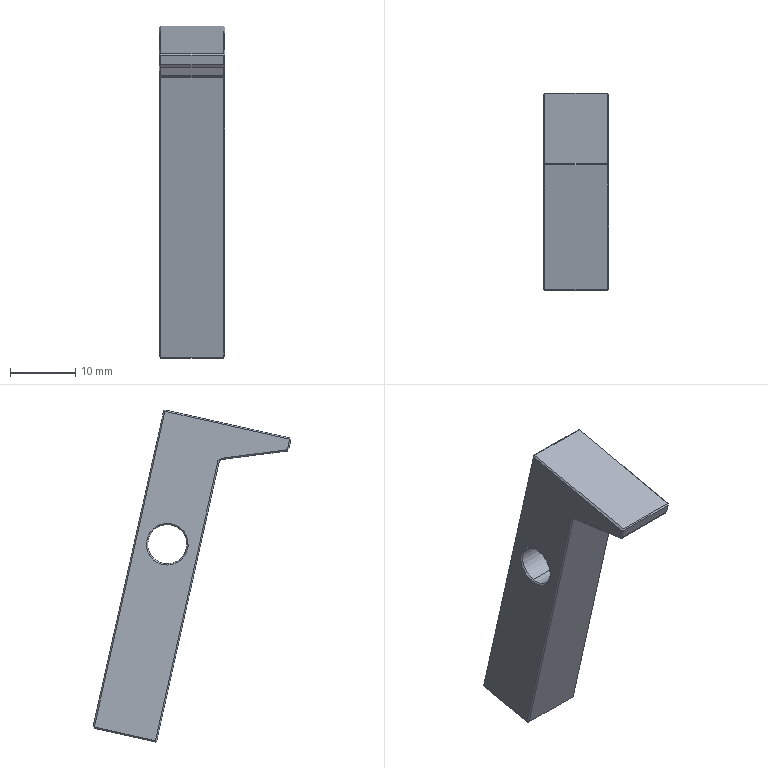Component | SolidWorks | PressJaw-1 | 1 solid | 44 faces | box 10 x 30.33 x 50.89 mm | volume 5092 mm3 | plane 36 | cone 4 | cylinder 2 | spline 2 | commonest cylinder face diameters 6 x2 | material 45
STEP:
#1=COLOUR_RGB('',0.7922,0.8196,0.9333);
#2=FILL_AREA_STYLE_COLOUR('',#1);
#3=FILL_AREA_STYLE('',(#2));
#4=SURFACE_STYLE_FILL_AREA(#3);
#5=SURFACE_SIDE_STYLE('',(#4));
#6=SURFACE_STYLE_USAGE(.BOTH.,#5);
#7=PRESENTATION_STYLE_ASSIGNMENT((#6));
#8=CARTESIAN_POINT('',(-14.809,1.597,40.726));
#9=VERTEX_POINT('',#8);
#10=CARTESIAN_POINT('',(-14.809,1.546,40.957));
#11=VERTEX_POINT('',#10);
#12=CARTESIAN_POINT('',(-14.809,1.571,40.842));
#13=DIRECTION('',(-1.,0.,0.));
#14=DIRECTION('',(0.,0.218,-0.9759));
#15=AXIS2_PLACEMENT_3D('',#12,#13,#14);
#16=CIRCLE('',#15,0.1181);
#17=EDGE_CURVE('',#9,#11,#16,.T.);
#18=ORIENTED_EDGE('',*,*,#17,.F.);
#19=CARTESIAN_POINT('',(-14.817,1.599,40.719));
#20=VERTEX_POINT('',#19);
#21=CARTESIAN_POINT('',(-14.809,1.597,40.726));
#22=DIRECTION('',(-0.7071,0.1542,-0.6901));
#23=VECTOR('',#22,39.37);
#24=LINE('',#21,#23);
#25=EDGE_CURVE('',#9,#20,#24,.T.);
#26=ORIENTED_EDGE('',*,*,#25,.T.);
#27=CARTESIAN_POINT('',(-14.817,1.544,40.965));
#28=VERTEX_POINT('',#27);
#29=CARTESIAN_POINT('',(-14.817,1.571,40.842));
#30=DIRECTION('',(1.,-0.,-0.));
#31=DIRECTION('',(0.,0.218,-0.9759));
#32=AXIS2_PLACEMENT_3D('',#29,#30,#31);
#33=CIRCLE('',#32,0.126);
#34=EDGE_CURVE('',#28,#20,#33,.T.);
#35=ORIENTED_EDGE('',*,*,#34,.F.);
#36=CARTESIAN_POINT('',(-14.809,1.546,40.957));
#37=DIRECTION('',(-0.7071,-0.1542,0.6901));
#38=VECTOR('',#37,39.37);
#39=LINE('',#36,#38);
#40=EDGE_CURVE('',#11,#28,#39,.T.);
#41=ORIENTED_EDGE('',*,*,#40,.F.);
#42=EDGE_LOOP('',(#18,#26,#35,#41));
#43=FACE_OUTER_BOUND('',#42,.T.);
#44=CARTESIAN_POINT('',(-14.809,1.571,40.842));
#45=DIRECTION('',(-1.,0.,0.));
#46=DIRECTION('',(0.,-0.218,0.9759));
#47=AXIS2_PLACEMENT_3D('',#44,#45,#46);
#48=CONICAL_SURFACE('',#47,0.1181,0.7854);
#49=ADVANCED_FACE('',(#43),#48,.F.);
#50=CARTESIAN_POINT('',(-14.431,1.546,40.957));
#51=VERTEX_POINT('',#50);
#52=CARTESIAN_POINT('',(-14.431,1.597,40.726));
#53=VERTEX_POINT('',#52);
#54=CARTESIAN_POINT('',(-14.431,1.571,40.842));
#55=DIRECTION('',(1.,-0.,-0.));
#56=DIRECTION('',(0.,0.218,-0.9759));
#57=AXIS2_PLACEMENT_3D('',#54,#55,#56);
#58=CIRCLE('',#57,0.1181);
#59=EDGE_CURVE('',#51,#53,#58,.T.);
#60=ORIENTED_EDGE('',*,*,#59,.F.);
#61=CARTESIAN_POINT('',(-14.424,1.544,40.965));
#62=VERTEX_POINT('',#61);
#63=CARTESIAN_POINT('',(-14.424,1.544,40.965));
#64=DIRECTION('',(0.7071,-0.1542,0.6901));
#65=VECTOR('',#64,39.37);
#66=LINE('',#63,#65);
#67=EDGE_CURVE('',#51,#62,#66,.T.);
#68=ORIENTED_EDGE('',*,*,#67,.T.);
#69=CARTESIAN_POINT('',(-14.424,1.599,40.719));
#70=VERTEX_POINT('',#69);
#71=CARTESIAN_POINT('',(-14.424,1.571,40.842));
#72=DIRECTION('',(-1.,0.,0.));
#73=DIRECTION('',(0.,0.218,-0.9759));
#74=AXIS2_PLACEMENT_3D('',#71,#72,#73);
#75=CIRCLE('',#74,0.126);
#76=EDGE_CURVE('',#70,#62,#75,.T.);
#77=ORIENTED_EDGE('',*,*,#76,.F.);
#78=CARTESIAN_POINT('',(-14.424,1.599,40.719));
#79=DIRECTION('',(0.7071,0.1542,-0.6901));
#80=VECTOR('',#79,39.37);
#81=LINE('',#78,#80);
#82=EDGE_CURVE('',#53,#70,#81,.T.);
#83=ORIENTED_EDGE('',*,*,#82,.F.);
#84=EDGE_LOOP('',(#60,#68,#77,#83));
#85=FACE_OUTER_BOUND('',#84,.T.);
#86=CARTESIAN_POINT('',(-14.424,1.571,40.842));
#87=DIRECTION('',(1.,-0.,-0.));
#88=DIRECTION('',(0.,0.218,-0.9759));
#89=AXIS2_PLACEMENT_3D('',#86,#87,#88);
#90=CONICAL_SURFACE('',#89,0.126,0.7854);
#91=ADVANCED_FACE('',(#85),#90,.F.);
#92=ORIENTED_EDGE('',*,*,#17,.T.);
#93=CARTESIAN_POINT('',(-14.817,1.546,40.957));
#94=DIRECTION('',(1.,-0.,-0.));
#95=VECTOR('',#94,39.37);
#96=LINE('',#93,#95);
#97=EDGE_CURVE('',#11,#51,#96,.T.);
#98=ORIENTED_EDGE('',*,*,#97,.T.);
#99=ORIENTED_EDGE('',*,*,#59,.T.);
#100=CARTESIAN_POINT('',(-14.817,1.597,40.726));
#101=DIRECTION('',(1.,-0.,-0.));
#102=VECTOR('',#101,39.37);
#103=LINE('',#100,#102);
#104=EDGE_CURVE('',#9,#53,#103,.T.);
#105=ORIENTED_EDGE('',*,*,#104,.F.);
#106=EDGE_LOOP('',(#92,#98,#99,#105));
#107=FACE_OUTER_BOUND('',#106,.T.);
#108=CARTESIAN_POINT('',(-14.817,1.571,40.842));
#109=DIRECTION('',(1.,-0.,-0.));
#110=DIRECTION('',(0.,0.218,-0.9759));
#111=AXIS2_PLACEMENT_3D('',#108,#109,#110);
#112=CYLINDRICAL_SURFACE('',#111,0.1181);
#113=ADVANCED_FACE('',(#107),#112,.F.);
#114=CARTESIAN_POINT('',(-14.817,1.244,41.36));
#115=VERTEX_POINT('',#114);
#116=CARTESIAN_POINT('',(-14.817,0.8471,41.412));
#117=VERTEX_POINT('',#116);
#118=CARTESIAN_POINT('',(-14.817,2.216,41.234));
#119=DIRECTION('',(-0.,-0.9917,0.1289));
#120=VECTOR('',#119,39.37);
#121=LINE('',#118,#120);
#122=EDGE_CURVE('',#115,#117,#121,.T.);
#123=ORIENTED_EDGE('',*,*,#122,.T.);
#124=CARTESIAN_POINT('',(-14.817,0.8328,41.475));
#125=VERTEX_POINT('',#124);
#126=CARTESIAN_POINT('',(-14.817,1.26,39.562));
#127=DIRECTION('',(0.,-0.218,0.9759));
#128=VECTOR('',#127,39.37);
#129=LINE('',#126,#128);
#130=EDGE_CURVE('',#117,#125,#129,.T.);
#131=ORIENTED_EDGE('',*,*,#130,.T.);
#132=CARTESIAN_POINT('',(-14.817,1.586,41.644));
#133=VERTEX_POINT('',#132);
#134=CARTESIAN_POINT('',(-14.817,1.594,41.645));
#135=DIRECTION('',(0.,0.9759,0.218));
#136=VECTOR('',#135,39.37);
#137=LINE('',#134,#136);
#138=EDGE_CURVE('',#125,#133,#137,.T.);
#139=ORIENTED_EDGE('',*,*,#138,.T.);
#140=CARTESIAN_POINT('',(-14.817,2.012,39.738));
#141=VERTEX_POINT('',#140);
#142=CARTESIAN_POINT('',(-14.817,2.013,39.73));
#143=DIRECTION('',(-0.,0.218,-0.9759));
#144=VECTOR('',#143,39.37);
#145=LINE('',#142,#144);
#146=EDGE_CURVE('',#133,#141,#145,.T.);
#147=ORIENTED_EDGE('',*,*,#146,.T.);
#148=CARTESIAN_POINT('',(-14.817,1.643,39.655));
#149=VERTEX_POINT('',#148);
#150=CARTESIAN_POINT('',(-14.817,2.019,39.74));
#151=DIRECTION('',(-0.,-0.9759,-0.218));
#152=VECTOR('',#151,39.37);
#153=LINE('',#150,#152);
#154=EDGE_CURVE('',#141,#149,#153,.T.);
#155=ORIENTED_EDGE('',*,*,#154,.T.);
#156=CARTESIAN_POINT('',(-14.817,1.265,41.344));
#157=VERTEX_POINT('',#156);
#158=CARTESIAN_POINT('',(-14.817,1.645,39.648));
#159=DIRECTION('',(0.,-0.218,0.9759));
#160=VECTOR('',#159,39.37);
#161=LINE('',#158,#160);
#162=EDGE_CURVE('',#149,#157,#161,.T.);
#163=ORIENTED_EDGE('',*,*,#162,.T.);
#164=CARTESIAN_POINT('',(-14.817,1.244,41.36));
#165=CARTESIAN_POINT('',(-14.817,1.265,41.344));
#166=B_SPLINE_CURVE_WITH_KNOTS('',1,(#164,#165),.UNSPECIFIED.,.F.,.F.,(2,2),(0.,0.0006718),.UNSPECIFIED.);
#167=EDGE_CURVE('',#115,#157,#166,.T.);
#168=ORIENTED_EDGE('',*,*,#167,.F.);
#169=EDGE_LOOP('',(#123,#131,#139,#147,#155,#163,#168));
#170=FACE_OUTER_BOUND('',#169,.T.);
#171=ORIENTED_EDGE('',*,*,#34,.T.);
#172=CARTESIAN_POINT('',(-14.817,1.571,40.842));
#173=DIRECTION('',(1.,-0.,-0.));
#174=DIRECTION('',(0.,0.218,-0.9759));
#175=AXIS2_PLACEMENT_3D('',#172,#173,#174);
#176=CIRCLE('',#175,0.126);
#177=EDGE_CURVE('',#20,#28,#176,.T.);
#178=ORIENTED_EDGE('',*,*,#177,.T.);
#179=EDGE_LOOP('',(#171,#178));
#180=FACE_BOUND('',#179,.T.);
#181=CARTESIAN_POINT('',(-14.817,2.021,39.732));
#182=DIRECTION('',(1.,-0.,-0.));
#183=DIRECTION('',(-0.,0.218,-0.9759));
#184=AXIS2_PLACEMENT_3D('',#181,#182,#183);
#185=PLANE('',#184);
#186=ADVANCED_FACE('',(#170,#180),#185,.F.);
#187=CARTESIAN_POINT('',(-14.424,2.012,39.738));
#188=VERTEX_POINT('',#187);
#189=CARTESIAN_POINT('',(-14.424,1.586,41.644));
#190=VERTEX_POINT('',#189);
#191=CARTESIAN_POINT('',(-14.424,1.584,41.651));
#192=DIRECTION('',(0.,-0.218,0.9759));
#193=VECTOR('',#192,39.37);
#194=LINE('',#191,#193);
#195=EDGE_CURVE('',#188,#190,#194,.T.);
#196=ORIENTED_EDGE('',*,*,#195,.T.);
#197=CARTESIAN_POINT('',(-14.424,0.8328,41.475));
#198=VERTEX_POINT('',#197);
#199=CARTESIAN_POINT('',(-14.424,0.8251,41.474));
#200=DIRECTION('',(-0.,-0.9759,-0.218));
#201=VECTOR('',#200,39.37);
#202=LINE('',#199,#201);
#203=EDGE_CURVE('',#190,#198,#202,.T.);
#204=ORIENTED_EDGE('',*,*,#203,.T.);
#205=CARTESIAN_POINT('',(-14.424,0.8471,41.412));
#206=VERTEX_POINT('',#205);
#207=CARTESIAN_POINT('',(-14.424,0.8483,41.406));
#208=DIRECTION('',(-0.,0.218,-0.9759));
#209=VECTOR('',#208,39.37);
#210=LINE('',#207,#209);
#211=EDGE_CURVE('',#198,#206,#210,.T.);
#212=ORIENTED_EDGE('',*,*,#211,.T.);
#213=CARTESIAN_POINT('',(-14.424,1.244,41.36));
#214=VERTEX_POINT('',#213);
#215=CARTESIAN_POINT('',(-14.424,1.257,41.358));
#216=DIRECTION('',(0.,0.9917,-0.1289));
#217=VECTOR('',#216,39.37);
#218=LINE('',#215,#217);
#219=EDGE_CURVE('',#206,#214,#218,.T.);
#220=ORIENTED_EDGE('',*,*,#219,.T.);
#221=CARTESIAN_POINT('',(-14.424,1.265,41.344));
#222=VERTEX_POINT('',#221);
#223=CARTESIAN_POINT('',(-14.424,1.265,41.344));
#224=CARTESIAN_POINT('',(-14.424,1.244,41.36));
#225=B_SPLINE_CURVE_WITH_KNOTS('',1,(#223,#224),.UNSPECIFIED.,.F.,.F.,(2,2),(0.,0.0006718),.UNSPECIFIED.);
#226=EDGE_CURVE('',#222,#214,#225,.T.);
#227=ORIENTED_EDGE('',*,*,#226,.F.);
#228=CARTESIAN_POINT('',(-14.424,1.643,39.655));
#229=VERTEX_POINT('',#228);
#230=CARTESIAN_POINT('',(-14.424,1.645,39.648));
#231=DIRECTION('',(-0.,0.218,-0.9759));
#232=VECTOR('',#231,39.37);
#233=LINE('',#230,#232);
#234=EDGE_CURVE('',#222,#229,#233,.T.);
#235=ORIENTED_EDGE('',*,*,#234,.T.);
#236=CARTESIAN_POINT('',(-14.424,2.019,39.74));
#237=DIRECTION('',(0.,0.9759,0.218));
#238=VECTOR('',#237,39.37);
#239=LINE('',#236,#238);
#240=EDGE_CURVE('',#229,#188,#239,.T.);
#241=ORIENTED_EDGE('',*,*,#240,.T.);
#242=EDGE_LOOP('',(#196,#204,#212,#220,#227,#235,#241));
#243=FACE_OUTER_BOUND('',#242,.T.);
#244=ORIENTED_EDGE('',*,*,#76,.T.);
#245=CARTESIAN_POINT('',(-14.424,1.571,40.842));
#246=DIRECTION('',(-1.,0.,0.));
#247=DIRECTION('',(0.,0.218,-0.9759));
#248=AXIS2_PLACEMENT_3D('',#245,#246,#247);
#249=CIRCLE('',#248,0.126);
#250=EDGE_CURVE('',#62,#70,#249,.T.);
#251=ORIENTED_EDGE('',*,*,#250,.T.);
#252=EDGE_LOOP('',(#244,#251));
#253=FACE_BOUND('',#252,.T.);
#254=CARTESIAN_POINT('',(-14.424,2.021,39.732));
#255=DIRECTION('',(1.,-0.,-0.));
#256=DIRECTION('',(-0.,0.218,-0.9759));
#257=AXIS2_PLACEMENT_3D('',#254,#255,#256);
#258=PLANE('',#257);
#259=ADVANCED_FACE('',(#243,#253),#258,.T.);
#260=CARTESIAN_POINT('',(-14.809,1.645,39.648));
#261=VERTEX_POINT('',#260);
#262=CARTESIAN_POINT('',(-14.809,2.013,39.73));
#263=VERTEX_POINT('',#262);
#264=CARTESIAN_POINT('',(-14.809,1.637,39.646));
#265=DIRECTION('',(0.,0.9759,0.218));
#266=VECTOR('',#265,39.37);
#267=LINE('',#264,#266);
#268=EDGE_CURVE('',#261,#263,#267,.T.);
#269=ORIENTED_EDGE('',*,*,#268,.T.);
#270=CARTESIAN_POINT('',(-14.431,2.013,39.73));
#271=VERTEX_POINT('',#270);
#272=CARTESIAN_POINT('',(-14.817,2.013,39.73));
#273=DIRECTION('',(1.,-0.,-0.));
#274=VECTOR('',#273,39.37);
#275=LINE('',#272,#274);
#276=EDGE_CURVE('',#263,#271,#275,.T.);
#277=ORIENTED_EDGE('',*,*,#276,.T.);
#278=CARTESIAN_POINT('',(-14.431,1.645,39.648));
#279=VERTEX_POINT('',#278);
#280=CARTESIAN_POINT('',(-14.431,1.637,39.646));
#281=DIRECTION('',(-0.,-0.9759,-0.218));
#282=VECTOR('',#281,39.37);
#283=LINE('',#280,#282);
#284=EDGE_CURVE('',#271,#279,#283,.T.);
#285=ORIENTED_EDGE('',*,*,#284,.T.);
#286=CARTESIAN_POINT('',(-14.817,1.645,39.648));
#287=DIRECTION('',(-1.,0.,0.));
#288=VECTOR('',#287,39.37);
#289=LINE('',#286,#288);
#290=EDGE_CURVE('',#279,#261,#289,.T.);
#291=ORIENTED_EDGE('',*,*,#290,.T.);
#292=EDGE_LOOP('',(#269,#277,#285,#291));
#293=FACE_OUTER_BOUND('',#292,.T.);
#294=CARTESIAN_POINT('',(-14.817,1.637,39.646));
#295=DIRECTION('',(0.,-0.218,0.9759));
#296=DIRECTION('',(1.,-0.,-0.));
#297=AXIS2_PLACEMENT_3D('',#294,#295,#296);
#298=PLANE('',#297);
#299=ADVANCED_FACE('',(#293),#298,.F.);
#300=CARTESIAN_POINT('',(-14.431,1.635,39.654));
#301=VERTEX_POINT('',#300);
#302=CARTESIAN_POINT('',(-14.431,1.258,41.343));
#303=VERTEX_POINT('',#302);
#304=CARTESIAN_POINT('',(-14.431,1.256,41.35));
#305=DIRECTION('',(0.,-0.218,0.9759));
#306=VECTOR('',#305,39.37);
#307=LINE('',#304,#306);
#308=EDGE_CURVE('',#301,#303,#307,.T.);
#309=ORIENTED_EDGE('',*,*,#308,.T.);
#310=CARTESIAN_POINT('',(-14.809,1.258,41.343));
#311=VERTEX_POINT('',#310);
#312=CARTESIAN_POINT('',(-14.817,1.258,41.343));
#313=DIRECTION('',(-1.,0.,0.));
#314=VECTOR('',#313,39.37);
#315=LINE('',#312,#314);
#316=EDGE_CURVE('',#303,#311,#315,.T.);
#317=ORIENTED_EDGE('',*,*,#316,.T.);
#318=CARTESIAN_POINT('',(-14.809,1.635,39.654));
#319=VERTEX_POINT('',#318);
#320=CARTESIAN_POINT('',(-14.809,1.256,41.35));
#321=DIRECTION('',(-0.,0.218,-0.9759));
#322=VECTOR('',#321,39.37);
#323=LINE('',#320,#322);
#324=EDGE_CURVE('',#311,#319,#323,.T.);
#325=ORIENTED_EDGE('',*,*,#324,.T.);
#326=CARTESIAN_POINT('',(-14.817,1.635,39.654));
#327=DIRECTION('',(1.,-0.,-0.));
#328=VECTOR('',#327,39.37);
#329=LINE('',#326,#328);
#330=EDGE_CURVE('',#319,#301,#329,.T.);
#331=ORIENTED_EDGE('',*,*,#330,.T.);
#332=EDGE_LOOP('',(#309,#317,#325,#331));
#333=FACE_OUTER_BOUND('',#332,.T.);
#334=CARTESIAN_POINT('',(-14.817,1.256,41.35));
#335=DIRECTION('',(0.,0.9759,0.218));
#336=DIRECTION('',(-0.,0.218,-0.9759));
#337=AXIS2_PLACEMENT_3D('',#334,#335,#336);
#338=PLANE('',#337);
#339=ADVANCED_FACE('',(#333),#338,.F.);
#340=CARTESIAN_POINT('',(-14.431,0.8484,41.403));
#341=VERTEX_POINT('',#340);
#342=CARTESIAN_POINT('',(-14.809,0.8484,41.403));
#343=VERTEX_POINT('',#342);
#344=CARTESIAN_POINT('',(-14.817,0.8484,41.403));
#345=DIRECTION('',(-1.,0.,0.));
#346=VECTOR('',#345,39.37);
#347=LINE('',#344,#346);
#348=EDGE_CURVE('',#341,#343,#347,.T.);
#349=ORIENTED_EDGE('',*,*,#348,.T.);
#350=CARTESIAN_POINT('',(-14.809,1.243,41.352));
#351=VERTEX_POINT('',#350);
#352=CARTESIAN_POINT('',(-14.809,0.8406,41.404));
#353=DIRECTION('',(0.,0.9917,-0.1289));
#354=VECTOR('',#353,39.37);
#355=LINE('',#352,#354);
#356=EDGE_CURVE('',#343,#351,#355,.T.);
#357=ORIENTED_EDGE('',*,*,#356,.T.);
#358=CARTESIAN_POINT('',(-14.431,1.243,41.352));
#359=VERTEX_POINT('',#358);
#360=CARTESIAN_POINT('',(-14.424,1.243,41.352));
#361=DIRECTION('',(1.,-0.,-0.));
#362=VECTOR('',#361,39.37);
#363=LINE('',#360,#362);
#364=EDGE_CURVE('',#351,#359,#363,.T.);
#365=ORIENTED_EDGE('',*,*,#364,.T.);
#366=CARTESIAN_POINT('',(-14.431,0.8406,41.404));
#367=DIRECTION('',(-0.,-0.9917,0.1289));
#368=VECTOR('',#367,39.37);
#369=LINE('',#366,#368);
#370=EDGE_CURVE('',#359,#341,#369,.T.);
#371=ORIENTED_EDGE('',*,*,#370,.T.);
#372=EDGE_LOOP('',(#349,#357,#365,#371));
#373=FACE_OUTER_BOUND('',#372,.T.);
#374=CARTESIAN_POINT('',(-14.817,0.8406,41.404));
#375=DIRECTION('',(0.,0.1289,0.9917));
#376=DIRECTION('',(0.,0.9917,-0.1289));
#377=AXIS2_PLACEMENT_3D('',#374,#375,#376);
#378=PLANE('',#377);
#379=ADVANCED_FACE('',(#373),#378,.F.);
#380=CARTESIAN_POINT('',(-14.809,0.8251,41.474));
#381=VERTEX_POINT('',#380);
#382=CARTESIAN_POINT('',(-14.809,0.8377,41.417));
#383=VERTEX_POINT('',#382);
#384=CARTESIAN_POINT('',(-14.809,0.8234,41.481));
#385=DIRECTION('',(-0.,0.218,-0.9759));
#386=VECTOR('',#385,39.37);
#387=LINE('',#384,#386);
#388=EDGE_CURVE('',#381,#383,#387,.T.);
#389=ORIENTED_EDGE('',*,*,#388,.T.);
#390=CARTESIAN_POINT('',(-14.431,0.8377,41.417));
#391=VERTEX_POINT('',#390);
#392=CARTESIAN_POINT('',(-14.817,0.8377,41.417));
#393=DIRECTION('',(1.,-0.,-0.));
#394=VECTOR('',#393,39.37);
#395=LINE('',#392,#394);
#396=EDGE_CURVE('',#383,#391,#395,.T.);
#397=ORIENTED_EDGE('',*,*,#396,.T.);
#398=CARTESIAN_POINT('',(-14.431,0.8251,41.474));
#399=VERTEX_POINT('',#398);
#400=CARTESIAN_POINT('',(-14.431,0.8234,41.481));
#401=DIRECTION('',(0.,-0.218,0.9759));
#402=VECTOR('',#401,39.37);
#403=LINE('',#400,#402);
#404=EDGE_CURVE('',#391,#399,#403,.T.);
#405=ORIENTED_EDGE('',*,*,#404,.T.);
#406=CARTESIAN_POINT('',(-14.817,0.8251,41.474));
#407=DIRECTION('',(-1.,0.,0.));
#408=VECTOR('',#407,39.37);
#409=LINE('',#406,#408);
#410=EDGE_CURVE('',#399,#381,#409,.T.);
#411=ORIENTED_EDGE('',*,*,#410,.T.);
#412=EDGE_LOOP('',(#389,#397,#405,#411));
#413=FACE_OUTER_BOUND('',#412,.T.);
#414=CARTESIAN_POINT('',(-14.817,0.8234,41.481));
#415=DIRECTION('',(0.,0.9759,0.218));
#416=DIRECTION('',(-1.,0.,0.));
#417=AXIS2_PLACEMENT_3D('',#414,#415,#416);
#418=PLANE('',#417);
#419=ADVANCED_FACE('',(#413),#418,.F.);
#420=CARTESIAN_POINT('',(-14.431,1.584,41.651));
#421=VERTEX_POINT('',#420);
#422=CARTESIAN_POINT('',(-14.809,1.584,41.651));
#423=VERTEX_POINT('',#422);
#424=CARTESIAN_POINT('',(-14.817,1.584,41.651));
#425=DIRECTION('',(-1.,0.,0.));
#426=VECTOR('',#425,39.37);
#427=LINE('',#424,#426);
#428=EDGE_CURVE('',#421,#423,#427,.T.);
#429=ORIENTED_EDGE('',*,*,#428,.T.);
#430=CARTESIAN_POINT('',(-14.809,0.8311,41.483));
#431=VERTEX_POINT('',#430);
#432=CARTESIAN_POINT('',(-14.809,1.592,41.653));
#433=DIRECTION('',(-0.,-0.9759,-0.218));
#434=VECTOR('',#433,39.37);
#435=LINE('',#432,#434);
#436=EDGE_CURVE('',#423,#431,#435,.T.);
#437=ORIENTED_EDGE('',*,*,#436,.T.);
#438=CARTESIAN_POINT('',(-14.431,0.8311,41.483));
#439=VERTEX_POINT('',#438);
#440=CARTESIAN_POINT('',(-14.817,0.8311,41.483));
#441=DIRECTION('',(1.,-0.,-0.));
#442=VECTOR('',#441,39.37);
#443=LINE('',#440,#442);
#444=EDGE_CURVE('',#431,#439,#443,.T.);
#445=ORIENTED_EDGE('',*,*,#444,.T.);
#446=CARTESIAN_POINT('',(-14.431,1.592,41.653));
#447=DIRECTION('',(0.,0.9759,0.218));
#448=VECTOR('',#447,39.37);
#449=LINE('',#446,#448);
#450=EDGE_CURVE('',#439,#421,#449,.T.);
#451=ORIENTED_EDGE('',*,*,#450,.T.);
#452=EDGE_LOOP('',(#429,#437,#445,#451));
#453=FACE_OUTER_BOUND('',#452,.T.);
#454=CARTESIAN_POINT('',(-14.817,1.592,41.653));
#455=DIRECTION('',(-0.,0.218,-0.9759));
#456=DIRECTION('',(-1.,0.,0.));
#457=AXIS2_PLACEMENT_3D('',#454,#455,#456);
#458=PLANE('',#457);
#459=ADVANCED_FACE('',(#453),#458,.F.);
#460=CARTESIAN_POINT('',(-14.809,1.594,41.645));
#461=VERTEX_POINT('',#460);
#462=CARTESIAN_POINT('',(-14.431,1.594,41.645));
#463=VERTEX_POINT('',#462);
#464=CARTESIAN_POINT('',(-14.817,1.594,41.645));
#465=DIRECTION('',(1.,-0.,-0.));
#466=VECTOR('',#465,39.37);
#467=LINE('',#464,#466);
#468=EDGE_CURVE('',#461,#463,#467,.T.);
#469=ORIENTED_EDGE('',*,*,#468,.T.);
#470=CARTESIAN_POINT('',(-14.431,2.019,39.74));
#471=VERTEX_POINT('',#470);
#472=CARTESIAN_POINT('',(-14.431,2.021,39.732));
#473=DIRECTION('',(-0.,0.218,-0.9759));
#474=VECTOR('',#473,39.37);
#475=LINE('',#472,#474);
#476=EDGE_CURVE('',#463,#471,#475,.T.);
#477=ORIENTED_EDGE('',*,*,#476,.T.);
#478=CARTESIAN_POINT('',(-14.809,2.019,39.74));
#479=VERTEX_POINT('',#478);
#480=CARTESIAN_POINT('',(-14.817,2.019,39.74));
#481=DIRECTION('',(-1.,0.,0.));
#482=VECTOR('',#481,39.37);
#483=LINE('',#480,#482);
#484=EDGE_CURVE('',#471,#479,#483,.T.);
#485=ORIENTED_EDGE('',*,*,#484,.T.);
#486=CARTESIAN_POINT('',(-14.809,2.021,39.732));
#487=DIRECTION('',(0.,-0.218,0.9759));
#488=VECTOR('',#487,39.37);
#489=LINE('',#486,#488);
#490=EDGE_CURVE('',#479,#461,#489,.T.);
#491=ORIENTED_EDGE('',*,*,#490,.T.);
#492=EDGE_LOOP('',(#469,#477,#485,#491));
#493=FACE_OUTER_BOUND('',#492,.T.);
#494=CARTESIAN_POINT('',(-14.817,2.021,39.732));
#495=DIRECTION('',(-0.,-0.9759,-0.218));
#496=DIRECTION('',(1.,-0.,-0.));
#497=AXIS2_PLACEMENT_3D('',#494,#495,#496);
#498=PLANE('',#497);
#499=ADVANCED_FACE('',(#493),#498,.F.);
#500=ORIENTED_EDGE('',*,*,#97,.F.);
#501=CARTESIAN_POINT('',(-14.809,1.571,40.842));
#502=DIRECTION('',(-1.,0.,0.));
#503=DIRECTION('',(0.,0.218,-0.9759));
#504=AXIS2_PLACEMENT_3D('',#501,#502,#503);
#505=CIRCLE('',#504,0.1181);
#506=EDGE_CURVE('',#11,#9,#505,.T.);
#507=ORIENTED_EDGE('',*,*,#506,.T.);
#508=ORIENTED_EDGE('',*,*,#104,.T.);
#509=CARTESIAN_POINT('',(-14.431,1.571,40.842));
#510=DIRECTION('',(1.,-0.,-0.));
#511=DIRECTION('',(0.,0.218,-0.9759));
#512=AXIS2_PLACEMENT_3D('',#509,#510,#511);
#513=CIRCLE('',#512,0.1181);
#514=EDGE_CURVE('',#53,#51,#513,.T.);
#515=ORIENTED_EDGE('',*,*,#514,.T.);
#516=EDGE_LOOP('',(#500,#507,#508,#515));
#517=FACE_OUTER_BOUND('',#516,.T.);
#518=CARTESIAN_POINT('',(-14.817,1.571,40.842));
#519=DIRECTION('',(1.,-0.,-0.));
#520=DIRECTION('',(0.,0.218,-0.9759));
#521=AXIS2_PLACEMENT_3D('',#518,#519,#520);
#522=CYLINDRICAL_SURFACE('',#521,0.1181);
#523=ADVANCED_FACE('',(#517),#522,.F.);
#524=ORIENTED_EDGE('',*,*,#67,.F.);
#525=ORIENTED_EDGE('',*,*,#514,.F.);
#526=ORIENTED_EDGE('',*,*,#82,.T.);
#527=ORIENTED_EDGE('',*,*,#250,.F.);
#528=EDGE_LOOP('',(#524,#525,#526,#527));
#529=FACE_OUTER_BOUND('',#528,.T.);
#530=CARTESIAN_POINT('',(-14.424,1.571,40.842));
#531=DIRECTION('',(1.,-0.,-0.));
#532=DIRECTION('',(0.,0.218,-0.9759));
#533=AXIS2_PLACEMENT_3D('',#530,#531,#532);
#534=CONICAL_SURFACE('',#533,0.126,0.7854);
#535=ADVANCED_FACE('',(#529),#534,.F.);
#536=ORIENTED_EDGE('',*,*,#25,.F.);
#537=ORIENTED_EDGE('',*,*,#506,.F.);
#538=ORIENTED_EDGE('',*,*,#40,.T.);
#539=ORIENTED_EDGE('',*,*,#177,.F.);
#540=EDGE_LOOP('',(#536,#537,#538,#539));
#541=FACE_OUTER_BOUND('',#540,.T.);
#542=CARTESIAN_POINT('',(-14.809,1.571,40.842));
#543=DIRECTION('',(-1.,0.,0.));
#544=DIRECTION('',(0.,-0.218,0.9759));
#545=AXIS2_PLACEMENT_3D('',#542,#543,#544);
#546=CONICAL_SURFACE('',#545,0.1181,0.7854);
#547=ADVANCED_FACE('',(#541),#546,.F.);
#548=CARTESIAN_POINT('',(-14.809,2.019,39.74));
#549=DIRECTION('',(-0.,-0.5359,-0.8443));
#550=VECTOR('',#549,39.37);
#551=LINE('',#548,#550);
#552=EDGE_CURVE('',#479,#263,#551,.T.);
#553=ORIENTED_EDGE('',*,*,#552,.F.);
#554=ORIENTED_EDGE('',*,*,#484,.F.);
#555=CARTESIAN_POINT('',(-14.431,2.013,39.73));
#556=DIRECTION('',(-0.,0.5359,0.8443));
#557=VECTOR('',#556,39.37);
#558=LINE('',#555,#557);
#559=EDGE_CURVE('',#271,#471,#558,.T.);
#560=ORIENTED_EDGE('',*,*,#559,.F.);
#561=ORIENTED_EDGE('',*,*,#276,.F.);
#562=EDGE_LOOP('',(#553,#554,#560,#561));
#563=FACE_OUTER_BOUND('',#562,.T.);
#564=CARTESIAN_POINT('',(-14.817,2.013,39.73));
#565=DIRECTION('',(-0.,-0.8443,0.5359));
#566=DIRECTION('',(1.,-0.,-0.));
#567=AXIS2_PLACEMENT_3D('',#564,#565,#566);
#568=PLANE('',#567);
#569=ADVANCED_FACE('',(#563),#568,.F.);
#570=CARTESIAN_POINT('',(-14.809,2.019,39.74));
#571=DIRECTION('',(-0.7071,-0.6901,-0.1542));
#572=VECTOR('',#571,39.37);
#573=LINE('',#570,#572);
#574=EDGE_CURVE('',#479,#141,#573,.T.);
#575=ORIENTED_EDGE('',*,*,#574,.F.);
#576=ORIENTED_EDGE('',*,*,#552,.T.);
#577=CARTESIAN_POINT('',(-14.813,2.013,39.734));
#578=DIRECTION('',(0.7071,0.1542,-0.6901));
#579=VECTOR('',#578,39.37);
#580=LINE('',#577,#579);
#581=EDGE_CURVE('',#141,#263,#580,.T.);
#582=ORIENTED_EDGE('',*,*,#581,.F.);
#583=EDGE_LOOP('',(#575,#576,#582));
#584=FACE_OUTER_BOUND('',#583,.T.);
#585=CARTESIAN_POINT('',(-14.809,2.019,39.74));
#586=DIRECTION('',(-0.5774,0.6893,-0.4376));
#587=DIRECTION('',(-0.,-0.5359,-0.8443));
#588=AXIS2_PLACEMENT_3D('',#585,#586,#587);
#589=PLANE('',#588);
#590=ADVANCED_FACE('',(#584),#589,.T.);
#591=CARTESIAN_POINT('',(-14.431,2.013,39.73));
#592=DIRECTION('',(0.7071,-0.1542,0.6901));
#593=VECTOR('',#592,39.37);
#594=LINE('',#591,#593);
#595=EDGE_CURVE('',#271,#188,#594,.T.);
#596=ORIENTED_EDGE('',*,*,#595,.F.);
#597=ORIENTED_EDGE('',*,*,#559,.T.);
#598=CARTESIAN_POINT('',(-14.428,2.016,39.739));
#599=DIRECTION('',(-0.7071,0.6901,0.1542));
#600=VECTOR('',#599,39.37);
#601=LINE('',#598,#600);
#602=EDGE_CURVE('',#188,#471,#601,.T.);
#603=ORIENTED_EDGE('',*,*,#602,.F.);
#604=EDGE_LOOP('',(#596,#597,#603));
#605=FACE_OUTER_BOUND('',#604,.T.);
#606=CARTESIAN_POINT('',(-14.431,2.013,39.73));
#607=DIRECTION('',(0.5774,0.6893,-0.4376));
#608=DIRECTION('',(-0.7071,0.6901,0.1542));
#609=AXIS2_PLACEMENT_3D('',#606,#607,#608);
#610=PLANE('',#609);
#611=ADVANCED_FACE('',(#605),#610,.T.);
#612=ORIENTED_EDGE('',*,*,#581,.T.);
#613=ORIENTED_EDGE('',*,*,#268,.F.);
#614=CARTESIAN_POINT('',(-14.813,1.644,39.652));
#615=DIRECTION('',(0.7071,0.1542,-0.6901));
#616=VECTOR('',#615,39.37);
#617=LINE('',#614,#616);
#618=EDGE_CURVE('',#149,#261,#617,.T.);
#619=ORIENTED_EDGE('',*,*,#618,.F.);
#620=ORIENTED_EDGE('',*,*,#154,.F.);
#621=EDGE_LOOP('',(#612,#613,#619,#620));
#622=FACE_OUTER_BOUND('',#621,.T.);
#623=CARTESIAN_POINT('',(-14.817,2.019,39.74));
#624=DIRECTION('',(0.7071,-0.1542,0.6901));
#625=DIRECTION('',(-0.,-0.9759,-0.218));
#626=AXIS2_PLACEMENT_3D('',#623,#624,#625);
#627=PLANE('',#626);
#628=ADVANCED_FACE('',(#622),#627,.F.);
#629=ORIENTED_EDGE('',*,*,#574,.T.);
#630=ORIENTED_EDGE('',*,*,#146,.F.);
#631=CARTESIAN_POINT('',(-14.817,1.586,41.644));
#632=DIRECTION('',(-0.7071,-0.6901,-0.1542));
#633=VECTOR('',#632,39.37);
#634=LINE('',#631,#633);
#635=EDGE_CURVE('',#461,#133,#634,.T.);
#636=ORIENTED_EDGE('',*,*,#635,.F.);
#637=ORIENTED_EDGE('',*,*,#490,.F.);
#638=EDGE_LOOP('',(#629,#630,#636,#637));
#639=FACE_OUTER_BOUND('',#638,.T.);
#640=CARTESIAN_POINT('',(-14.817,2.013,39.73));
#641=DIRECTION('',(0.7071,-0.6901,-0.1542));
#642=DIRECTION('',(-0.,0.218,-0.9759));
#643=AXIS2_PLACEMENT_3D('',#640,#641,#642);
#644=PLANE('',#643);
#645=ADVANCED_FACE('',(#639),#644,.F.);
#646=CARTESIAN_POINT('',(-14.431,1.594,41.645));
#647=DIRECTION('',(0.,-0.8443,0.5359));
#648=VECTOR('',#647,39.37);
#649=LINE('',#646,#648);
#650=EDGE_CURVE('',#463,#421,#649,.T.);
#651=ORIENTED_EDGE('',*,*,#650,.F.);
#652=ORIENTED_EDGE('',*,*,#468,.F.);
#653=CARTESIAN_POINT('',(-14.809,1.589,41.648));
#654=DIRECTION('',(-0.,0.8443,-0.5359));
#655=VECTOR('',#654,39.37);
#656=LINE('',#653,#655);
#657=EDGE_CURVE('',#423,#461,#656,.T.);
#658=ORIENTED_EDGE('',*,*,#657,.F.);
#659=ORIENTED_EDGE('',*,*,#428,.F.);
#660=EDGE_LOOP('',(#651,#652,#658,#659));
#661=FACE_OUTER_BOUND('',#660,.T.);
#662=CARTESIAN_POINT('',(-14.817,1.594,41.645));
#663=DIRECTION('',(-0.,-0.5359,-0.8443));
#664=DIRECTION('',(1.,-0.,-0.));
#665=AXIS2_PLACEMENT_3D('',#662,#663,#664);
#666=PLANE('',#665);
#667=ADVANCED_FACE('',(#661),#666,.F.);
#668=ORIENTED_EDGE('',*,*,#602,.T.);
#669=ORIENTED_EDGE('',*,*,#476,.F.);
#670=CARTESIAN_POINT('',(-14.431,1.594,41.645));
#671=DIRECTION('',(-0.7071,0.6901,0.1542));
#672=VECTOR('',#671,39.37);
#673=LINE('',#670,#672);
#674=EDGE_CURVE('',#190,#463,#673,.T.);
#675=ORIENTED_EDGE('',*,*,#674,.F.);
#676=ORIENTED_EDGE('',*,*,#195,.F.);
#677=EDGE_LOOP('',(#668,#669,#675,#676));
#678=FACE_OUTER_BOUND('',#677,.T.);
#679=CARTESIAN_POINT('',(-14.431,2.021,39.732));
#680=DIRECTION('',(0.7071,0.6901,0.1542));
#681=DIRECTION('',(0.,-0.218,0.9759));
#682=AXIS2_PLACEMENT_3D('',#679,#680,#681);
#683=PLANE('',#682);
#684=ADVANCED_FACE('',(#678),#683,.T.);
#685=ORIENTED_EDGE('',*,*,#595,.T.);
#686=ORIENTED_EDGE('',*,*,#240,.F.);
#687=CARTESIAN_POINT('',(-14.424,1.643,39.655));
#688=DIRECTION('',(0.7071,-0.1542,0.6901));
#689=VECTOR('',#688,39.37);
#690=LINE('',#687,#689);
#691=EDGE_CURVE('',#279,#229,#690,.T.);
#692=ORIENTED_EDGE('',*,*,#691,.F.);
#693=ORIENTED_EDGE('',*,*,#284,.F.);
#694=EDGE_LOOP('',(#685,#686,#692,#693));
#695=FACE_OUTER_BOUND('',#694,.T.);
#696=CARTESIAN_POINT('',(-14.431,1.637,39.646));
#697=DIRECTION('',(0.7071,0.1542,-0.6901));
#698=DIRECTION('',(0.,0.9759,0.218));
#699=AXIS2_PLACEMENT_3D('',#696,#697,#698);
#700=PLANE('',#699);
#701=ADVANCED_FACE('',(#695),#700,.T.);
#702=CARTESIAN_POINT('',(-14.809,1.635,39.654));
#703=DIRECTION('',(0.,-0.8443,0.5359));
#704=VECTOR('',#703,39.37);
#705=LINE('',#702,#704);
#706=EDGE_CURVE('',#261,#319,#705,.T.);
#707=ORIENTED_EDGE('',*,*,#706,.F.);
#708=ORIENTED_EDGE('',*,*,#290,.F.);
#709=CARTESIAN_POINT('',(-14.431,1.64,39.651));
#710=DIRECTION('',(-0.,0.8443,-0.5359));
#711=VECTOR('',#710,39.37);
#712=LINE('',#709,#711);
#713=EDGE_CURVE('',#301,#279,#712,.T.);
#714=ORIENTED_EDGE('',*,*,#713,.F.);
#715=ORIENTED_EDGE('',*,*,#330,.F.);
#716=EDGE_LOOP('',(#707,#708,#714,#715));
#717=FACE_OUTER_BOUND('',#716,.T.);
#718=CARTESIAN_POINT('',(-14.817,1.635,39.654));
#719=DIRECTION('',(0.,0.5359,0.8443));
#720=DIRECTION('',(1.,-0.,-0.));
#721=AXIS2_PLACEMENT_3D('',#718,#719,#720);
#722=PLANE('',#721);
#723=ADVANCED_FACE('',(#717),#722,.F.);
#724=ORIENTED_EDGE('',*,*,#618,.T.);
#725=ORIENTED_EDGE('',*,*,#706,.T.);
#726=CARTESIAN_POINT('',(-14.809,1.635,39.654));
#727=DIRECTION('',(0.7071,-0.6901,-0.1542));
#728=VECTOR('',#727,39.37);
#729=LINE('',#726,#728);
#730=EDGE_CURVE('',#149,#319,#729,.T.);
#731=ORIENTED_EDGE('',*,*,#730,.F.);
#732=EDGE_LOOP('',(#724,#725,#731));
#733=FACE_OUTER_BOUND('',#732,.T.);
#734=CARTESIAN_POINT('',(-14.809,1.635,39.654));
#735=DIRECTION('',(-0.5774,-0.4376,-0.6893));
#736=DIRECTION('',(-0.,-0.8443,0.5359));
#737=AXIS2_PLACEMENT_3D('',#734,#735,#736);
#738=PLANE('',#737);
#739=ADVANCED_FACE('',(#733),#738,.T.);
#740=ORIENTED_EDGE('',*,*,#657,.T.);
#741=ORIENTED_EDGE('',*,*,#635,.T.);
#742=CARTESIAN_POINT('',(-14.817,1.586,41.644));
#743=DIRECTION('',(-0.7071,0.1542,-0.6901));
#744=VECTOR('',#743,39.37);
#745=LINE('',#742,#744);
#746=EDGE_CURVE('',#423,#133,#745,.T.);
#747=ORIENTED_EDGE('',*,*,#746,.F.);
#748=EDGE_LOOP('',(#740,#741,#747));
#749=FACE_OUTER_BOUND('',#748,.T.);
#750=CARTESIAN_POINT('',(-14.817,1.586,41.644));
#751=DIRECTION('',(-0.5774,0.4376,0.6893));
#752=DIRECTION('',(0.,0.8443,-0.5359));
#753=AXIS2_PLACEMENT_3D('',#750,#751,#752);
#754=PLANE('',#753);
#755=ADVANCED_FACE('',(#749),#754,.T.);
#756=ORIENTED_EDGE('',*,*,#674,.T.);
#757=ORIENTED_EDGE('',*,*,#650,.T.);
#758=CARTESIAN_POINT('',(-14.428,1.585,41.647));
#759=DIRECTION('',(-0.7071,-0.1542,0.6901));
#760=VECTOR('',#759,39.37);
#761=LINE('',#758,#760);
#762=EDGE_CURVE('',#190,#421,#761,.T.);
#763=ORIENTED_EDGE('',*,*,#762,.F.);
#764=EDGE_LOOP('',(#756,#757,#763));
#765=FACE_OUTER_BOUND('',#764,.T.);
#766=CARTESIAN_POINT('',(-14.431,1.594,41.645));
#767=DIRECTION('',(0.5774,0.4376,0.6893));
#768=DIRECTION('',(-0.7071,0.6901,0.1542));
#769=AXIS2_PLACEMENT_3D('',#766,#767,#768);
#770=PLANE('',#769);
#771=ADVANCED_FACE('',(#765),#770,.T.);
#772=ORIENTED_EDGE('',*,*,#713,.T.);
#773=ORIENTED_EDGE('',*,*,#691,.T.);
#774=CARTESIAN_POINT('',(-14.424,1.643,39.655));
#775=DIRECTION('',(0.7071,0.6901,0.1542));
#776=VECTOR('',#775,39.37);
#777=LINE('',#774,#776);
#778=EDGE_CURVE('',#301,#229,#777,.T.);
#779=ORIENTED_EDGE('',*,*,#778,.F.);
#780=EDGE_LOOP('',(#772,#773,#779));
#781=FACE_OUTER_BOUND('',#780,.T.);
#782=CARTESIAN_POINT('',(-14.424,1.643,39.655));
#783=DIRECTION('',(0.5774,-0.4376,-0.6893));
#784=DIRECTION('',(-0.7071,0.1542,-0.6901));
#785=AXIS2_PLACEMENT_3D('',#782,#783,#784);
#786=PLANE('',#785);
#787=ADVANCED_FACE('',(#781),#786,.T.);
#788=ORIENTED_EDGE('',*,*,#730,.T.);
#789=ORIENTED_EDGE('',*,*,#324,.F.);
#790=CARTESIAN_POINT('',(-14.817,1.265,41.344));
#791=DIRECTION('',(0.7071,-0.6901,-0.1542));
#792=VECTOR('',#791,39.37);
#793=LINE('',#790,#792);
#794=EDGE_CURVE('',#157,#311,#793,.T.);
#795=ORIENTED_EDGE('',*,*,#794,.F.);
#796=ORIENTED_EDGE('',*,*,#162,.F.);
#797=EDGE_LOOP('',(#788,#789,#795,#796));
#798=FACE_OUTER_BOUND('',#797,.T.);
#799=CARTESIAN_POINT('',(-14.817,1.645,39.648));
#800=DIRECTION('',(0.7071,0.6901,0.1542));
#801=DIRECTION('',(0.,-0.218,0.9759));
#802=AXIS2_PLACEMENT_3D('',#799,#800,#801);
#803=PLANE('',#802);
#804=ADVANCED_FACE('',(#798),#803,.F.);
#805=ORIENTED_EDGE('',*,*,#746,.T.);
#806=ORIENTED_EDGE('',*,*,#138,.F.);
#807=CARTESIAN_POINT('',(-14.809,0.8311,41.483));
#808=DIRECTION('',(-0.7071,0.1542,-0.6901));
#809=VECTOR('',#808,39.37);
#810=LINE('',#807,#809);
#811=EDGE_CURVE('',#431,#125,#810,.T.);
#812=ORIENTED_EDGE('',*,*,#811,.F.);
#813=ORIENTED_EDGE('',*,*,#436,.F.);
#814=EDGE_LOOP('',(#805,#806,#812,#813));
#815=FACE_OUTER_BOUND('',#814,.T.);
#816=CARTESIAN_POINT('',(-14.817,1.594,41.645));
#817=DIRECTION('',(0.7071,0.1542,-0.6901));
#818=DIRECTION('',(0.,0.9759,0.218));
#819=AXIS2_PLACEMENT_3D('',#816,#817,#818);
#820=PLANE('',#819);
#821=ADVANCED_FACE('',(#815),#820,.F.);
#822=CARTESIAN_POINT('',(-14.431,0.8281,41.478));
#823=DIRECTION('',(-0.,-0.5359,-0.8443));
#824=VECTOR('',#823,39.37);
#825=LINE('',#822,#824);
#826=EDGE_CURVE('',#439,#399,#825,.T.);
#827=ORIENTED_EDGE('',*,*,#826,.F.);
#828=ORIENTED_EDGE('',*,*,#444,.F.);
#829=CARTESIAN_POINT('',(-14.809,0.8311,41.483));
#830=DIRECTION('',(0.,0.5359,0.8443));
#831=VECTOR('',#830,39.37);
#832=LINE('',#829,#831);
#833=EDGE_CURVE('',#381,#431,#832,.T.);
#834=ORIENTED_EDGE('',*,*,#833,.F.);
#835=ORIENTED_EDGE('',*,*,#410,.F.);
#836=EDGE_LOOP('',(#827,#828,#834,#835));
#837=FACE_OUTER_BOUND('',#836,.T.);
#838=CARTESIAN_POINT('',(-14.817,0.8311,41.483));
#839=DIRECTION('',(0.,0.8443,-0.5359));
#840=DIRECTION('',(1.,-0.,-0.));
#841=AXIS2_PLACEMENT_3D('',#838,#839,#840);
#842=PLANE('',#841);
#843=ADVANCED_FACE('',(#837),#842,.F.);
#844=ORIENTED_EDGE('',*,*,#762,.T.);
#845=ORIENTED_EDGE('',*,*,#450,.F.);
#846=CARTESIAN_POINT('',(-14.424,0.8328,41.475));
#847=DIRECTION('',(-0.7071,-0.1542,0.6901));
#848=VECTOR('',#847,39.37);
#849=LINE('',#846,#848);
#850=EDGE_CURVE('',#198,#439,#849,.T.);
#851=ORIENTED_EDGE('',*,*,#850,.F.);
#852=ORIENTED_EDGE('',*,*,#203,.F.);
#853=EDGE_LOOP('',(#844,#845,#851,#852));
#854=FACE_OUTER_BOUND('',#853,.T.);
#855=CARTESIAN_POINT('',(-14.431,1.592,41.653));
#856=DIRECTION('',(0.7071,-0.1542,0.6901));
#857=DIRECTION('',(-0.,-0.9759,-0.218));
#858=AXIS2_PLACEMENT_3D('',#855,#856,#857);
#859=PLANE('',#858);
#860=ADVANCED_FACE('',(#854),#859,.T.);
#861=ORIENTED_EDGE('',*,*,#778,.T.);
#862=ORIENTED_EDGE('',*,*,#234,.F.);
#863=CARTESIAN_POINT('',(-14.431,1.258,41.343));
#864=DIRECTION('',(0.7071,0.6901,0.1542));
#865=VECTOR('',#864,39.37);
#866=LINE('',#863,#865);
#867=EDGE_CURVE('',#303,#222,#866,.T.);
#868=ORIENTED_EDGE('',*,*,#867,.F.);
#869=ORIENTED_EDGE('',*,*,#308,.F.);
#870=EDGE_LOOP('',(#861,#862,#868,#869));
#871=FACE_OUTER_BOUND('',#870,.T.);
#872=CARTESIAN_POINT('',(-14.431,1.256,41.35));
#873=DIRECTION('',(0.7071,-0.6901,-0.1542));
#874=DIRECTION('',(-0.,0.218,-0.9759));
#875=AXIS2_PLACEMENT_3D('',#872,#873,#874);
#876=PLANE('',#875);
#877=ADVANCED_FACE('',(#871),#876,.T.);
#878=CARTESIAN_POINT('',(-14.809,1.258,41.343));
#879=CARTESIAN_POINT('',(-14.809,1.243,41.352));
#880=B_SPLINE_CURVE_WITH_KNOTS('',1,(#878,#879),.UNSPECIFIED.,.F.,.F.,(2,2),(0.,0.0004447),.UNSPECIFIED.);
#881=EDGE_CURVE('',#311,#351,#880,.T.);
#882=ORIENTED_EDGE('',*,*,#881,.F.);
#883=ORIENTED_EDGE('',*,*,#316,.F.);
#884=CARTESIAN_POINT('',(-14.431,1.243,41.352));
#885=CARTESIAN_POINT('',(-14.431,1.258,41.343));
#886=B_SPLINE_CURVE_WITH_KNOTS('',1,(#884,#885),.UNSPECIFIED.,.F.,.F.,(2,2),(0.,0.0004447),.UNSPECIFIED.);
#887=EDGE_CURVE('',#359,#303,#886,.T.);
#888=ORIENTED_EDGE('',*,*,#887,.F.);
#889=ORIENTED_EDGE('',*,*,#364,.F.);
#890=EDGE_LOOP('',(#882,#883,#888,#889));
#891=FACE_OUTER_BOUND('',#890,.T.);
#892=CARTESIAN_POINT('',(-14.817,1.243,41.352));
#893=DIRECTION('',(-0.,-0.5359,-0.8443));
#894=DIRECTION('',(-1.,0.,0.));
#895=AXIS2_PLACEMENT_3D('',#892,#893,#894);
#896=PLANE('',#895);
#897=ADVANCED_FACE('',(#891),#896,.T.);
#898=ORIENTED_EDGE('',*,*,#794,.T.);
#899=ORIENTED_EDGE('',*,*,#881,.T.);
#900=CARTESIAN_POINT('',(-14.809,1.243,41.352));
#901=DIRECTION('',(0.7071,-0.09114,-0.7012));
#902=VECTOR('',#901,39.37);
#903=LINE('',#900,#902);
#904=EDGE_CURVE('',#115,#351,#903,.T.);
#905=ORIENTED_EDGE('',*,*,#904,.F.);
#906=ORIENTED_EDGE('',*,*,#167,.T.);
#907=EDGE_LOOP('',(#898,#899,#905,#906));
#908=FACE_OUTER_BOUND('',#907,.T.);
#909=CARTESIAN_POINT('',(-14.809,1.243,41.352));
#910=CARTESIAN_POINT('',(-14.809,1.258,41.343));
#911=CARTESIAN_POINT('',(-14.817,1.244,41.36));
#912=CARTESIAN_POINT('',(-14.817,1.265,41.344));
#913=B_SPLINE_SURFACE_WITH_KNOTS('',1,1,((#909,#910),(#911,#912)),.UNSPECIFIED.,.F.,.F.,.F.,(2,2),(2,2),(0.,1.),(0.,1.),.UNSPECIFIED.);
#914=ADVANCED_FACE('',(#908),#913,.T.);
#915=ORIENTED_EDGE('',*,*,#833,.T.);
#916=ORIENTED_EDGE('',*,*,#811,.T.);
#917=CARTESIAN_POINT('',(-14.813,0.829,41.474));
#918=DIRECTION('',(-0.7071,0.6901,0.1542));
#919=VECTOR('',#918,39.37);
#920=LINE('',#917,#919);
#921=EDGE_CURVE('',#381,#125,#920,.T.);
#922=ORIENTED_EDGE('',*,*,#921,.F.);
#923=EDGE_LOOP('',(#915,#916,#922));
#924=FACE_OUTER_BOUND('',#923,.T.);
#925=CARTESIAN_POINT('',(-14.809,0.8311,41.483));
#926=DIRECTION('',(-0.5774,-0.6893,0.4376));
#927=DIRECTION('',(0.,0.5359,0.8443));
#928=AXIS2_PLACEMENT_3D('',#925,#926,#927);
#929=PLANE('',#928);
#930=ADVANCED_FACE('',(#924),#929,.T.);
#931=ORIENTED_EDGE('',*,*,#850,.T.);
#932=ORIENTED_EDGE('',*,*,#826,.T.);
#933=CARTESIAN_POINT('',(-14.424,0.8328,41.475));
#934=DIRECTION('',(-0.7071,-0.6901,-0.1542));
#935=VECTOR('',#934,39.37);
#936=LINE('',#933,#935);
#937=EDGE_CURVE('',#198,#399,#936,.T.);
#938=ORIENTED_EDGE('',*,*,#937,.F.);
#939=EDGE_LOOP('',(#931,#932,#938));
#940=FACE_OUTER_BOUND('',#939,.T.);
#941=CARTESIAN_POINT('',(-14.424,0.8328,41.475));
#942=DIRECTION('',(0.5774,-0.6893,0.4376));
#943=DIRECTION('',(0.7071,0.6901,0.1542));
#944=AXIS2_PLACEMENT_3D('',#941,#942,#943);
#945=PLANE('',#944);
#946=ADVANCED_FACE('',(#940),#945,.T.);
#947=ORIENTED_EDGE('',*,*,#867,.T.);
#948=ORIENTED_EDGE('',*,*,#226,.T.);
#949=CARTESIAN_POINT('',(-14.424,1.244,41.36));
#950=DIRECTION('',(0.7071,0.09114,0.7012));
#951=VECTOR('',#950,39.37);
#952=LINE('',#949,#951);
#953=EDGE_CURVE('',#359,#214,#952,.T.);
#954=ORIENTED_EDGE('',*,*,#953,.F.);
#955=ORIENTED_EDGE('',*,*,#887,.T.);
#956=EDGE_LOOP('',(#947,#948,#954,#955));
#957=FACE_OUTER_BOUND('',#956,.T.);
#958=CARTESIAN_POINT('',(-14.431,1.258,41.343));
#959=CARTESIAN_POINT('',(-14.431,1.243,41.352));
#960=CARTESIAN_POINT('',(-14.424,1.265,41.344));
#961=CARTESIAN_POINT('',(-14.424,1.244,41.36));
#962=B_SPLINE_SURFACE_WITH_KNOTS('',1,1,((#958,#959),(#960,#961)),.UNSPECIFIED.,.F.,.F.,.F.,(2,2),(2,2),(0.,1.),(0.,1.),.UNSPECIFIED.);
#963=ADVANCED_FACE('',(#957),#962,.T.);
#964=ORIENTED_EDGE('',*,*,#904,.T.);
#965=ORIENTED_EDGE('',*,*,#356,.F.);
#966=CARTESIAN_POINT('',(-14.809,0.8484,41.403));
#967=DIRECTION('',(0.6917,0.1165,-0.7127));
#968=VECTOR('',#967,39.37);
#969=LINE('',#966,#968);
#970=EDGE_CURVE('',#117,#343,#969,.T.);
#971=ORIENTED_EDGE('',*,*,#970,.F.);
#972=ORIENTED_EDGE('',*,*,#122,.F.);
#973=EDGE_LOOP('',(#964,#965,#971,#972));
#974=FACE_OUTER_BOUND('',#973,.T.);
#975=CARTESIAN_POINT('',(-14.817,2.216,41.234));
#976=DIRECTION('',(0.7071,0.09114,0.7012));
#977=DIRECTION('',(-0.,-0.9917,0.1289));
#978=AXIS2_PLACEMENT_3D('',#975,#976,#977);
#979=PLANE('',#978);
#980=ADVANCED_FACE('',(#974),#979,.F.);
#981=ORIENTED_EDGE('',*,*,#921,.T.);
#982=ORIENTED_EDGE('',*,*,#130,.F.);
#983=CARTESIAN_POINT('',(-14.817,0.8469,41.412));
#984=DIRECTION('',(-0.5826,0.6921,-0.4261));
#985=VECTOR('',#984,39.37);
#986=LINE('',#983,#985);
#987=EDGE_CURVE('',#383,#117,#986,.T.);
#988=ORIENTED_EDGE('',*,*,#987,.F.);
#989=ORIENTED_EDGE('',*,*,#388,.F.);
#990=EDGE_LOOP('',(#981,#982,#988,#989));
#991=FACE_OUTER_BOUND('',#990,.T.);
#992=CARTESIAN_POINT('',(-14.817,1.26,39.562));
#993=DIRECTION('',(0.7071,0.6901,0.1542));
#994=DIRECTION('',(0.,-0.218,0.9759));
#995=AXIS2_PLACEMENT_3D('',#992,#993,#994);
#996=PLANE('',#995);
#997=ADVANCED_FACE('',(#991),#996,.F.);
#998=ORIENTED_EDGE('',*,*,#937,.T.);
#999=ORIENTED_EDGE('',*,*,#404,.F.);
#1000=CARTESIAN_POINT('',(-14.431,0.8377,41.417));
#1001=DIRECTION('',(-0.5826,-0.6921,0.4261));
#1002=VECTOR('',#1001,39.37);
#1003=LINE('',#1000,#1002);
#1004=EDGE_CURVE('',#206,#391,#1003,.T.);
#1005=ORIENTED_EDGE('',*,*,#1004,.F.);
#1006=ORIENTED_EDGE('',*,*,#211,.F.);
#1007=EDGE_LOOP('',(#998,#999,#1005,#1006));
#1008=FACE_OUTER_BOUND('',#1007,.T.);
#1009=CARTESIAN_POINT('',(-14.431,0.8234,41.481));
#1010=DIRECTION('',(0.7071,-0.6901,-0.1542));
#1011=DIRECTION('',(-0.,0.218,-0.9759));
#1012=AXIS2_PLACEMENT_3D('',#1009,#1010,#1011);
#1013=PLANE('',#1012);
#1014=ADVANCED_FACE('',(#1008),#1013,.T.);
#1015=ORIENTED_EDGE('',*,*,#953,.T.);
#1016=ORIENTED_EDGE('',*,*,#219,.F.);
#1017=CARTESIAN_POINT('',(-14.424,0.8471,41.411));
#1018=DIRECTION('',(0.6917,-0.1165,0.7127));
#1019=VECTOR('',#1018,39.37);
#1020=LINE('',#1017,#1019);
#1021=EDGE_CURVE('',#341,#206,#1020,.T.);
#1022=ORIENTED_EDGE('',*,*,#1021,.F.);
#1023=ORIENTED_EDGE('',*,*,#370,.F.);
#1024=EDGE_LOOP('',(#1015,#1016,#1022,#1023));
#1025=FACE_OUTER_BOUND('',#1024,.T.);
#1026=CARTESIAN_POINT('',(-14.431,0.8406,41.404));
#1027=DIRECTION('',(0.7071,-0.09114,-0.7012));
#1028=DIRECTION('',(0.,0.9917,-0.1289));
#1029=AXIS2_PLACEMENT_3D('',#1026,#1027,#1028);
#1030=PLANE('',#1029);
#1031=ADVANCED_FACE('',(#1025),#1030,.T.);
#1032=ORIENTED_EDGE('',*,*,#987,.T.);
#1033=ORIENTED_EDGE('',*,*,#970,.T.);
#1034=CARTESIAN_POINT('',(-14.809,0.8484,41.403));
#1035=DIRECTION('',(-0.,0.6101,-0.7924));
#1036=VECTOR('',#1035,39.37);
#1037=LINE('',#1034,#1036);
#1038=EDGE_CURVE('',#383,#343,#1037,.T.);
#1039=ORIENTED_EDGE('',*,*,#1038,.F.);
#1040=EDGE_LOOP('',(#1032,#1033,#1039));
#1041=FACE_OUTER_BOUND('',#1040,.T.);
#1042=CARTESIAN_POINT('',(-14.809,0.8484,41.403));
#1043=DIRECTION('',(-0.4437,-0.7101,-0.5467));
#1044=DIRECTION('',(0.8776,-0.4679,-0.1045));
#1045=AXIS2_PLACEMENT_3D('',#1042,#1043,#1044);
#1046=PLANE('',#1045);
#1047=ADVANCED_FACE('',(#1041),#1046,.T.);
#1048=ORIENTED_EDGE('',*,*,#1021,.T.);
#1049=ORIENTED_EDGE('',*,*,#1004,.T.);
#1050=CARTESIAN_POINT('',(-14.431,0.8377,41.417));
#1051=DIRECTION('',(0.,-0.6101,0.7924));
#1052=VECTOR('',#1051,39.37);
#1053=LINE('',#1050,#1052);
#1054=EDGE_CURVE('',#341,#391,#1053,.T.);
#1055=ORIENTED_EDGE('',*,*,#1054,.F.);
#1056=EDGE_LOOP('',(#1048,#1049,#1055));
#1057=FACE_OUTER_BOUND('',#1056,.T.);
#1058=CARTESIAN_POINT('',(-14.431,0.8377,41.417));
#1059=DIRECTION('',(0.4437,-0.7101,-0.5467));
#1060=DIRECTION('',(0.8776,0.4679,0.1045));
#1061=AXIS2_PLACEMENT_3D('',#1058,#1059,#1060);
#1062=PLANE('',#1061);
#1063=ADVANCED_FACE('',(#1057),#1062,.T.);
#1064=ORIENTED_EDGE('',*,*,#1038,.T.);
#1065=ORIENTED_EDGE('',*,*,#348,.F.);
#1066=ORIENTED_EDGE('',*,*,#1054,.T.);
#1067=ORIENTED_EDGE('',*,*,#396,.F.);
#1068=EDGE_LOOP('',(#1064,#1065,#1066,#1067));
#1069=FACE_OUTER_BOUND('',#1068,.T.);
#1070=CARTESIAN_POINT('',(-14.817,0.8377,41.417));
#1071=DIRECTION('',(0.,0.7924,0.6101));
#1072=DIRECTION('',(1.,-0.,-0.));
#1073=AXIS2_PLACEMENT_3D('',#1070,#1071,#1072);
#1074=PLANE('',#1073);
#1075=ADVANCED_FACE('',(#1069),#1074,.F.);
#1076=CLOSED_SHELL('',(#49,#91,#113,#186,#259,#299,#339,#379,#419,#459,#499,#523,#535,#547,#569,#590,#611,#628,#645,#667,#684,#701,#723,#739,#755,#771,#787,#804,#821,#843,#860,#877,#897,#914,#930,#946,#963,#980,#997,#1014,#1031,#1047,#1063,#1075));
#1077=MANIFOLD_SOLID_BREP('',#1076);
#1078=STYLED_ITEM('',(#7),#1077);
#1079=(LENGTH_UNIT()NAMED_UNIT(*)SI_UNIT($,.METRE.));
#1080=LENGTH_MEASURE_WITH_UNIT(LENGTH_MEASURE(0.0254),#1079);
#1081=DIMENSIONAL_EXPONENTS(1.,0.,0.,0.,0.,0.,0.);
#1082=(CONVERSION_BASED_UNIT('',#1080)LENGTH_UNIT()NAMED_UNIT(#1081));
#1083=UNCERTAINTY_MEASURE_WITH_UNIT(LENGTH_MEASURE(0.00001),#1082,'','');
#1084=(NAMED_UNIT(*)PLANE_ANGLE_UNIT()SI_UNIT($,.RADIAN.));
#1085=(NAMED_UNIT(*)SI_UNIT($,.STERADIAN.)SOLID_ANGLE_UNIT());
#1086=(GEOMETRIC_REPRESENTATION_CONTEXT(3)GLOBAL_UNCERTAINTY_ASSIGNED_CONTEXT((#1083))GLOBAL_UNIT_ASSIGNED_CONTEXT((#1082,#1084,#1085))REPRESENTATION_CONTEXT('',''));
#1087=MECHANICAL_DESIGN_GEOMETRIC_PRESENTATION_REPRESENTATION('',(#1078),#1086);
#1088=CARTESIAN_POINT('',(0.,0.,0.));
#1089=DIRECTION('',(0.,0.,1.));
#1090=DIRECTION('',(1.,0.,0.));
#1091=AXIS2_PLACEMENT_3D('',#1088,#1089,#1090);
#1092=(LENGTH_UNIT()NAMED_UNIT(*)SI_UNIT($,.METRE.));
#1093=LENGTH_MEASURE_WITH_UNIT(LENGTH_MEASURE(0.0254),#1092);
#1094=DIMENSIONAL_EXPONENTS(1.,0.,0.,0.,0.,0.,0.);
#1095=(CONVERSION_BASED_UNIT('',#1093)LENGTH_UNIT()NAMED_UNIT(#1094));
#1096=UNCERTAINTY_MEASURE_WITH_UNIT(LENGTH_MEASURE(0.00001),#1095,'','');
#1097=(NAMED_UNIT(*)PLANE_ANGLE_UNIT()SI_UNIT($,.RADIAN.));
#1098=(NAMED_UNIT(*)SI_UNIT($,.STERADIAN.)SOLID_ANGLE_UNIT());
#1099=(GEOMETRIC_REPRESENTATION_CONTEXT(3)GLOBAL_UNCERTAINTY_ASSIGNED_CONTEXT((#1096))GLOBAL_UNIT_ASSIGNED_CONTEXT((#1095,#1097,#1098))REPRESENTATION_CONTEXT('',''));
#1100=ADVANCED_BREP_SHAPE_REPRESENTATION('',(#1077,#1091),#1099);
#1101=PRESENTATION_LAYER_ASSIGNMENT('','',(#1078));